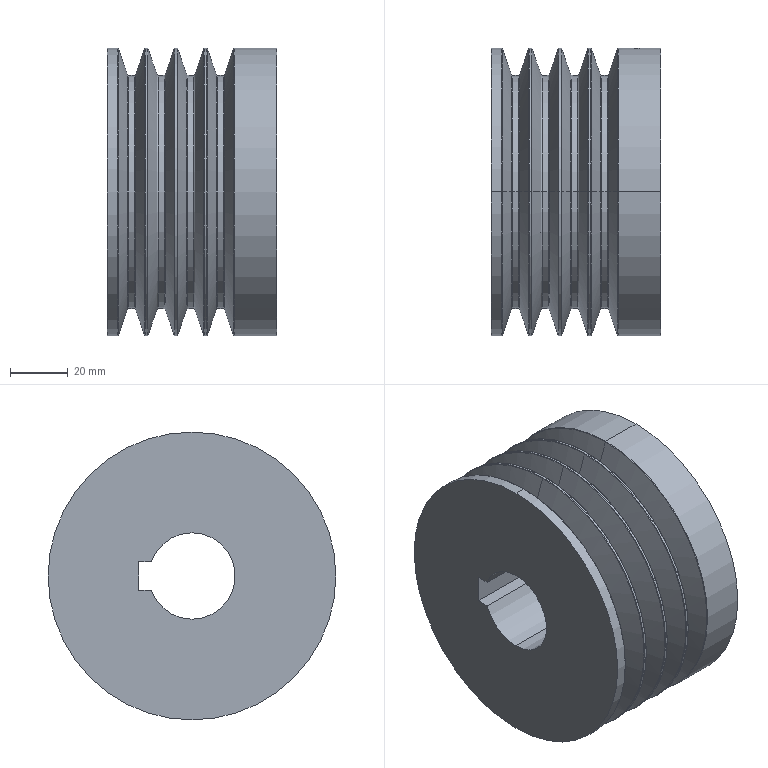Component | SolidWorks | SawBladeDrivePulley-2 | 1 solid | 76 faces | box 59 x 100 x 100 mm | volume 352620 mm3 | torus 32 | cylinder 23 | cone 16 | plane 5 | commonest cylinder face diameters 100 x10 81 x8 30 x3 6.8 x2
build123d program:
from build123d import *

# Parameters (mm, degrees)
FILLET2_R             = 5
SKETCH2_W             = 10
SKETCH2_H             = 7
CUT_EXTRUDE1_DEPTH    = 171.367
FILLET3_R             = 0.2
FILLET4_R             = 0.5
SKETCH3_R             = 105
CUT_EXTRUDE2_DEPTH    = 150.67
BOSS_EXTRUDE1_START   = 10
SKETCH4_R             = 50
BOSS_EXTRUDE1_DEPTH   = 10
M8_TAPPED_HOLE1_D     = 6.8
M8_TAPPED_HOLE1_DEPTH = 35
M8_TAPPED_HOLE1_TIP   = 2.043


with BuildPart() as part:
    # Sketch1 → Revolve1 (revolve)
    with BuildSketch(Plane.XY, mode=Mode.PRIVATE) as revolve1_sk:
        Polygon((0, 60), (0, 100), (46, 100), (46, 50), (49.86, 50), (53.131, 40.5), (55.829, 40.5), (59.1, 50), (60.16, 50), (63.431, 40.5), (66.129, 40.5), (69.4, 50), (70.46, 50), (73.731, 40.5), (76.429, 40.5), (79.7, 50), (80.76, 50), (84.031, 40.5), (86.729, 40.5), (90, 50), (95, 50), (95, 15), (15, 15), (15, 50), (15, 60), align=None)
    revolve(revolve1_sk.sketch.rotate(Axis((0, 0, 0), (1, 0, 0)), 90), axis=Axis((0, 0, 0), (1, 0, 0)))

    # Fillet2
    fillet2_edges = [part.edges().sort_by_distance(p)[0] for p in [
        (46, 0, -100),
        (0, 0, -100),
        (0, 0, -60),
    ]]
    fillet(fillet2_edges, radius=FILLET2_R)

    # Sketch2 → Cut-Extrude1 (cut, through all)
    with BuildSketch(Plane(origin=(95, 0, 0), x_dir=(0, 0, -1), z_dir=(1, 0, 0))):
        with Locations((0, 15)):
            Rectangle(SKETCH2_W, SKETCH2_H)
    extrude(amount=-CUT_EXTRUDE1_DEPTH, mode=Mode.SUBTRACT)

    # Fillet3
    fillet3_edges = [part.edges().sort_by_distance(p)[0] for p in [
        (90, 0, -50),
        (80.76, 0, -50),
        (79.7, 0, -50),
        (70.46, 0, -50),
        (69.4, 0, -50),
        (60.16, 0, -50),
        (59.1, 0, -50),
        (49.86, 0, -50),
    ]]
    fillet(fillet3_edges, radius=FILLET3_R)

    # Fillet4
    fillet4_edges = [part.edges().sort_by_distance(p)[0] for p in [
        (86.729, 0, -40.5),
        (84.031, 0, -40.5),
        (76.429, 0, -40.5),
        (73.731, 0, -40.5),
        (66.129, 0, -40.5),
        (63.431, 0, -40.5),
        (55.829, 0, -40.5),
        (53.131, 0, -40.5),
    ]]
    fillet(fillet4_edges, radius=FILLET4_R)

    # Sketch3 → Cut-Extrude2 (cut, through all)
    with BuildSketch(Plane(origin=(46, 0, 0), x_dir=(0, 0, -1), z_dir=(1, 0, 0))):
        Circle(SKETCH3_R)
    extrude(amount=-CUT_EXTRUDE2_DEPTH, mode=Mode.SUBTRACT)

    # Sketch4 → Boss-Extrude1 (add)
    with BuildSketch(Plane(origin=(95, 0, 0), x_dir=(0, 0, -1), z_dir=(1, 0, 0)).offset(BOSS_EXTRUDE1_START)):
        Circle(SKETCH4_R)
        with BuildLine():
            Line((5, 14.142), (5, 18.5))
            Line((5, 18.5), (-5, 18.5))
            Line((-5, 18.5), (-5, 14.142))
            ThreePointArc((-5, 14.142), (0, -15), (5, 14.142))
        make_face(mode=Mode.SUBTRACT)
    extrude(amount=-BOSS_EXTRUDE1_DEPTH)

    # M8 Tapped Hole1
    with Locations(Plane(origin=(97, 50, 0), x_dir=(0, 0, 1), z_dir=(0, 1, 0))):
        with Locations((0, 0)):
            Hole(M8_TAPPED_HOLE1_D / 2, depth=M8_TAPPED_HOLE1_DEPTH)
            with Locations((0, 0, -(M8_TAPPED_HOLE1_DEPTH + M8_TAPPED_HOLE1_TIP / 2))):  # 118° drill point
                Cone(0, M8_TAPPED_HOLE1_D / 2, M8_TAPPED_HOLE1_TIP, mode=Mode.SUBTRACT)


solid = part.part

# Placed as in the assembly
solid = solid.moved(Location((-617.309, -4.181, 0), (0, 0, 0)))